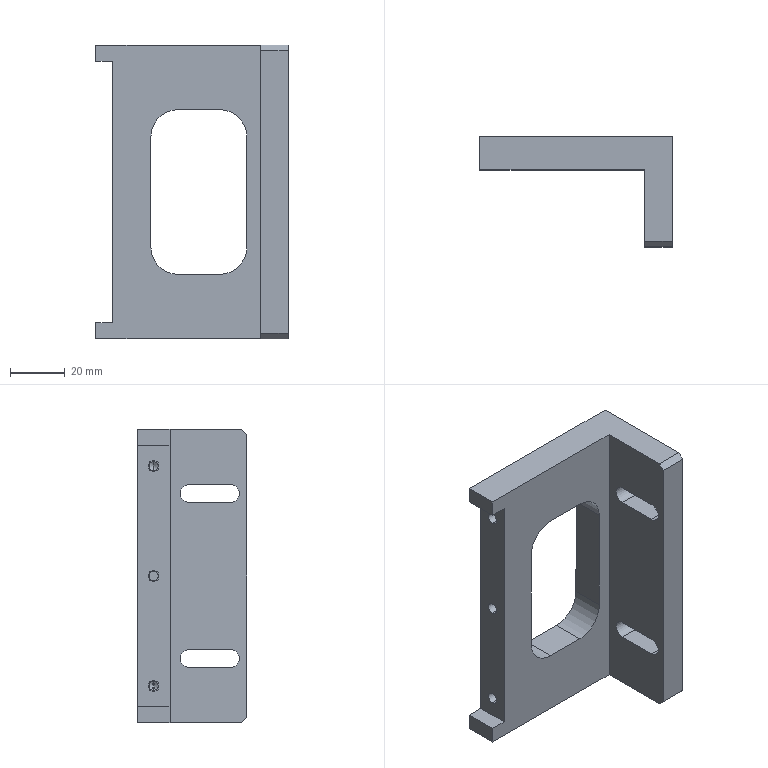Component | SolidWorks | F01AE00021-D54312B-1 | 1 solid | 49 faces | box 70 x 40 x 107 mm | volume 85638 mm3 | plane 25 | cylinder 20 | cone 4 | commonest cylinder face diameters 3.3 x6 4 x6 6.5 x4 20 x4 | material AL6061
build123d program:
from build123d import *

# Parameters (mm, degrees)
BOSS_EXTRUDE1_DEPTH           = 53.5
CHAMFER1_SIZE                 = 2
CUT_EXTRUDE1_DEPTH            = 50
SKETCH9_W                     = 95
SKETCH9_H                     = 6
CUT_EXTRUDE4_DEPTH            = 97.759
M4_TAPPED_HOLE1_D             = 3.3
M4_TAPPED_HOLE1_DEPTH         = 15
M4_TAPPED_HOLE1_TIP           = 0.9914
SKETCH8_W                     = 60
SKETCH8_H                     = 35
CUT_EXTRUDE3_DEPTH            = 97.759
FILLET2_R                     = 10
M4_THREADMAJORRELIEF_START    = 51
M4_THREADMAJORRELIEF_SKETCH_R = 2
M4_THREADMAJORRELIEF_DEPTH    = 13


with BuildPart() as part:
    # Sketch1 → Boss-Extrude1 (new, symmetric)
    with BuildSketch(Plane.XY):
        Polygon((0, 0), (0, 70), (12, 70), (12, 10), (40, 10), (40, 0), align=None)
    extrude(amount=BOSS_EXTRUDE1_DEPTH, both=True)

    # Chamfer1
    chamfer1_edges = [part.edges().sort_by_distance(p)[0] for p in [
        (40, 5, 53.5),
        (40, 5, -53.5),
    ]]
    chamfer(chamfer1_edges, length=CHAMFER1_SIZE)

    # Sketch2 → Cut-Extrude1 (cut)
    with BuildSketch(Plane(origin=(0, 10, 0), x_dir=(1, 0, 0), z_dir=(0, 1, 0))):
        with BuildLine():
            Line((19, 33.25), (34, 33.25))
            ThreePointArc((34, 33.25), (37.25, 30), (34, 26.75))
            Line((34, 26.75), (19, 26.75))
            ThreePointArc((19, 26.75), (15.75, 30), (19, 33.25))
        make_face()
        with BuildLine():
            Line((19, -33.25), (34, -33.25))
            ThreePointArc((34, -33.25), (37.25, -30), (34, -26.75))
            Line((34, -26.75), (19, -26.75))
            ThreePointArc((19, -26.75), (15.75, -30), (19, -33.25))
        make_face()
    extrude(amount=-CUT_EXTRUDE1_DEPTH, mode=Mode.SUBTRACT)

    # Sketch9 → Cut-Extrude4 (cut, through all)
    with BuildSketch(Plane.ZY):
        with Locations((0, 67)):
            Rectangle(SKETCH9_W, SKETCH9_H)
    extrude(amount=-CUT_EXTRUDE4_DEPTH, mode=Mode.SUBTRACT)

    # M4 Tapped Hole1
    with Locations(Plane(origin=(-21.337, 64, -8.571), x_dir=(1, 0, 0), z_dir=(0, 1, 0))):
        with Locations((27.337, -48.571), (27.337, -8.571), (27.337, 31.429)):
            Hole(M4_TAPPED_HOLE1_D / 2, depth=M4_TAPPED_HOLE1_DEPTH)
            with Locations((0, 0, -(M4_TAPPED_HOLE1_DEPTH + M4_TAPPED_HOLE1_TIP / 2))):  # 118° drill point
                Cone(0, M4_TAPPED_HOLE1_D / 2, M4_TAPPED_HOLE1_TIP, mode=Mode.SUBTRACT)

    # Sketch8 → Cut-Extrude3 (cut, through all)
    with BuildSketch(Plane.ZY):
        with Locations((0, 32.5)):
            Rectangle(SKETCH8_W, SKETCH8_H)
    extrude(amount=-CUT_EXTRUDE3_DEPTH, mode=Mode.SUBTRACT)

    # Fillet2
    fillet2_edges = [part.edges().sort_by_distance(p)[0] for p in [
        (6, 15, -30),
        (6, 50, 30),
        (6, 15, 30),
        (6, 50, -30),
    ]]
    fillet(fillet2_edges, radius=FILLET2_R)

    # M4_ThreadMajorRelief_Sketch → M4_ThreadMajorRelief (cut)
    with BuildSketch(Plane(origin=(0, 0, 0), x_dir=(1, 0, 0), z_dir=(0, 1, 0)).offset(M4_THREADMAJORRELIEF_START)):
        with Locations(Location((6, 0, 0), (0, 0, 90))):
            Circle(M4_THREADMAJORRELIEF_SKETCH_R)
        with Locations(Location((6, -40, 0), (0, 0, 90))):
            Circle(M4_THREADMAJORRELIEF_SKETCH_R)
        with Locations(Location((6, 40, 0), (0, 0, 90))):
            Circle(M4_THREADMAJORRELIEF_SKETCH_R)
    extrude(amount=M4_THREADMAJORRELIEF_DEPTH, mode=Mode.SUBTRACT)


solid = part.part

# Placed as in the assembly
solid = solid.moved(Location((354.434, 87.705, 246.764), (180, 0, 90)))